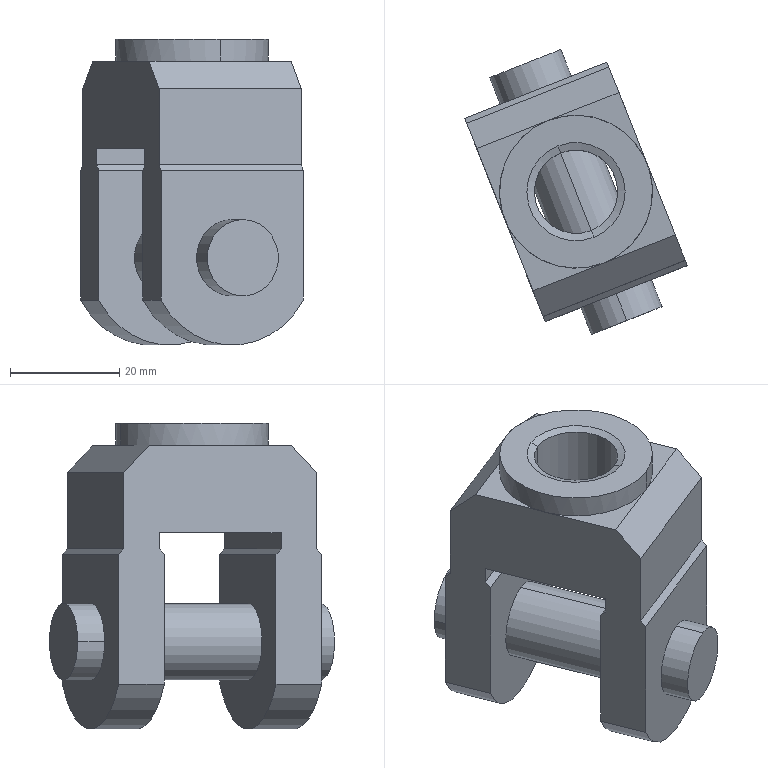Component | SolidWorks | Y-G05-1 | 1 solid | 38 faces | volume 36665 mm3 | plane 20 | cylinder 12 | spline 4 | cone 2 | commonest cylinder face diameters 14 x6 28 x2 15.29 x2 32 x2 | material Plain Carbon Steel